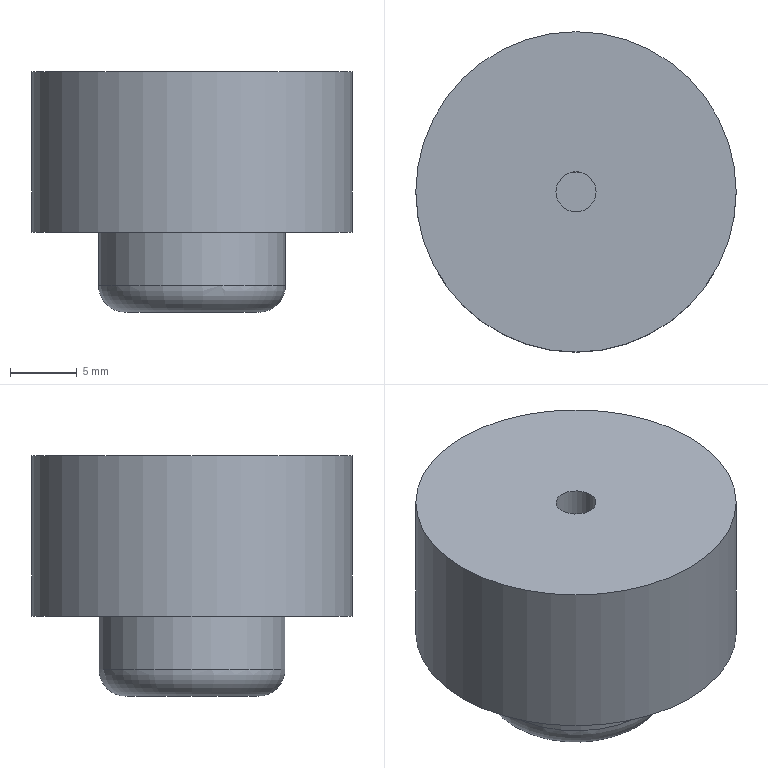Component | NX | MOTOR_MOUNT_3 | 1 solid | 8 faces | box 24 x 24 x 18 mm | volume 6275 mm3 | plane 4 | cylinder 3 | torus 1 | commonest cylinder face diameters 24 x1 14 x1 3 x1
STEP:
#1=CARTESIAN_POINT('',(0.,0.,0.));
#2=DIRECTION('',(0.,0.,1.));
#3=DIRECTION('',(1.,0.,0.));
#4=AXIS2_PLACEMENT_3D('',#1,#2,#3);
#5=CARTESIAN_POINT('',(92.558,84.858,-55.892));
#6=VERTEX_POINT('',#5);
#7=CARTESIAN_POINT('',(85.558,84.858,-55.892));
#8=DIRECTION('',(0.,0.,-1.));
#9=DIRECTION('',(1.,0.,0.));
#10=AXIS2_PLACEMENT_3D('',#7,#8,#9);
#11=CIRCLE('',#10,7.);
#12=CARTESIAN_POINT('',(85.558,84.858,-55.892));
#13=DIRECTION('',(0.,0.,-1.));
#14=DIRECTION('',(1.,0.,0.));
#15=AXIS2_PLACEMENT_3D('',#12,#13,#14);
#16=PLANE('',#15);
#17=CARTESIAN_POINT('',(0.,0.));
#18=DIRECTION('',(1.,0.));
#19=AXIS2_PLACEMENT_2D('',#17,#18);
#20=CIRCLE('',#19,7.);
#21=(GEOMETRIC_REPRESENTATION_CONTEXT(2)PARAMETRIC_REPRESENTATION_CONTEXT()REPRESENTATION_CONTEXT('',''));
#22=DEFINITIONAL_REPRESENTATION('',(#20),#21);
#23=PCURVE('',#16,#22);
#24=CARTESIAN_POINT('',(85.558,84.858,-55.892));
#25=DIRECTION('',(0.,0.,-1.));
#26=DIRECTION('',(1.,0.,0.));
#27=AXIS2_PLACEMENT_3D('',#24,#25,#26);
#28=CYLINDRICAL_SURFACE('',#27,7.);
#29=CARTESIAN_POINT('',(0.,0.));
#30=DIRECTION('',(1.,0.));
#31=VECTOR('',#30,1.);
#32=LINE('',#29,#31);
#33=(GEOMETRIC_REPRESENTATION_CONTEXT(2)PARAMETRIC_REPRESENTATION_CONTEXT()REPRESENTATION_CONTEXT('',''));
#34=DEFINITIONAL_REPRESENTATION('',(#32),#33);
#35=PCURVE('',#28,#34);
#36=SURFACE_CURVE('',#11,(#23,#35),.PCURVE_S1.);
#37=EDGE_CURVE('',#6,#6,#36,.T.);
#38=ORIENTED_EDGE('',*,*,#37,.F.);
#39=EDGE_LOOP('',(#38));
#40=FACE_BOUND('',#39,.T.);
#41=CARTESIAN_POINT('',(97.558,84.858,-55.892));
#42=VERTEX_POINT('',#41);
#43=CARTESIAN_POINT('',(85.558,84.858,-55.892));
#44=DIRECTION('',(0.,0.,1.));
#45=DIRECTION('',(1.,0.,0.));
#46=AXIS2_PLACEMENT_3D('',#43,#44,#45);
#47=CIRCLE('',#46,12.);
#48=CARTESIAN_POINT('',(12.,0.));
#49=CARTESIAN_POINT('',(12.,-20.785));
#50=CARTESIAN_POINT('',(-6.,-10.392));
#51=CARTESIAN_POINT('',(-24.,-0.));
#52=CARTESIAN_POINT('',(-6.,10.392));
#53=CARTESIAN_POINT('',(12.,20.785));
#54=CARTESIAN_POINT('',(12.,0.));
#55=(BOUNDED_CURVE()B_SPLINE_CURVE(2,(#48,#49,#50,#51,#52,#53,#54),.UNSPECIFIED.,.T.,.F.)B_SPLINE_CURVE_WITH_KNOTS((1,2,2,2,2,1),(-2.094,0.,2.094,4.189,6.283,8.378),.UNSPECIFIED.)CURVE()GEOMETRIC_REPRESENTATION_ITEM()RATIONAL_B_SPLINE_CURVE((1.,0.5,1.,0.5,1.,0.5,1.))REPRESENTATION_ITEM(''));
#56=(GEOMETRIC_REPRESENTATION_CONTEXT(2)PARAMETRIC_REPRESENTATION_CONTEXT()REPRESENTATION_CONTEXT('',''));
#57=DEFINITIONAL_REPRESENTATION('',(#55),#56);
#58=PCURVE('',#16,#57);
#59=CARTESIAN_POINT('',(85.558,84.858,-43.892));
#60=DIRECTION('',(0.,0.,-1.));
#61=DIRECTION('',(1.,0.,0.));
#62=AXIS2_PLACEMENT_3D('',#59,#60,#61);
#63=CYLINDRICAL_SURFACE('',#62,12.);
#64=CARTESIAN_POINT('',(6.283,12.));
#65=DIRECTION('',(-1.,0.));
#66=VECTOR('',#65,1.);
#67=LINE('',#64,#66);
#68=(GEOMETRIC_REPRESENTATION_CONTEXT(2)PARAMETRIC_REPRESENTATION_CONTEXT()REPRESENTATION_CONTEXT('',''));
#69=DEFINITIONAL_REPRESENTATION('',(#67),#68);
#70=PCURVE('',#63,#69);
#71=SURFACE_CURVE('',#47,(#58,#70),.PCURVE_S1.);
#72=EDGE_CURVE('',#42,#42,#71,.T.);
#73=ORIENTED_EDGE('',*,*,#72,.F.);
#74=EDGE_LOOP('',(#73));
#75=FACE_BOUND('',#74,.T.);
#76=ADVANCED_FACE('',(#40,#75),#16,.T.);
#77=CARTESIAN_POINT('',(87.058,84.858,-43.892));
#78=VERTEX_POINT('',#77);
#79=CARTESIAN_POINT('',(85.558,84.858,-43.892));
#80=DIRECTION('',(0.,0.,1.));
#81=DIRECTION('',(1.,0.,0.));
#82=AXIS2_PLACEMENT_3D('',#79,#80,#81);
#83=CIRCLE('',#82,1.5);
#84=CARTESIAN_POINT('',(85.558,84.858,-43.892));
#85=DIRECTION('',(0.,0.,1.));
#86=DIRECTION('',(-1.,0.,0.));
#87=AXIS2_PLACEMENT_3D('',#84,#85,#86);
#88=PLANE('',#87);
#89=CARTESIAN_POINT('',(0.,0.));
#90=DIRECTION('',(-1.,0.));
#91=AXIS2_PLACEMENT_2D('',#89,#90);
#92=CIRCLE('',#91,1.5);
#93=(GEOMETRIC_REPRESENTATION_CONTEXT(2)PARAMETRIC_REPRESENTATION_CONTEXT()REPRESENTATION_CONTEXT('',''));
#94=DEFINITIONAL_REPRESENTATION('',(#92),#93);
#95=PCURVE('',#88,#94);
#96=CARTESIAN_POINT('',(85.558,84.858,-49.892));
#97=DIRECTION('',(0.,0.,1.));
#98=DIRECTION('',(-1.,0.,0.));
#99=AXIS2_PLACEMENT_3D('',#96,#97,#98);
#100=CYLINDRICAL_SURFACE('',#99,1.5);
#101=CARTESIAN_POINT('',(3.142,6.));
#102=DIRECTION('',(1.,0.));
#103=VECTOR('',#102,1.);
#104=LINE('',#101,#103);
#105=(GEOMETRIC_REPRESENTATION_CONTEXT(2)PARAMETRIC_REPRESENTATION_CONTEXT()REPRESENTATION_CONTEXT('',''));
#106=DEFINITIONAL_REPRESENTATION('',(#104),#105);
#107=PCURVE('',#100,#106);
#108=SURFACE_CURVE('',#83,(#95,#107),.PCURVE_S1.);
#109=EDGE_CURVE('',#78,#78,#108,.T.);
#110=ORIENTED_EDGE('',*,*,#109,.F.);
#111=EDGE_LOOP('',(#110));
#112=FACE_BOUND('',#111,.T.);
#113=CARTESIAN_POINT('',(97.558,84.858,-43.892));
#114=VERTEX_POINT('',#113);
#115=CARTESIAN_POINT('',(85.558,84.858,-43.892));
#116=DIRECTION('',(0.,0.,-1.));
#117=DIRECTION('',(1.,0.,0.));
#118=AXIS2_PLACEMENT_3D('',#115,#116,#117);
#119=CIRCLE('',#118,12.);
#120=CARTESIAN_POINT('',(-12.,0.));
#121=CARTESIAN_POINT('',(-12.,20.785));
#122=CARTESIAN_POINT('',(6.,10.392));
#123=CARTESIAN_POINT('',(24.,0.));
#124=CARTESIAN_POINT('',(6.,-10.392));
#125=CARTESIAN_POINT('',(-12.,-20.785));
#126=CARTESIAN_POINT('',(-12.,0.));
#127=(BOUNDED_CURVE()B_SPLINE_CURVE(2,(#120,#121,#122,#123,#124,#125,#126),.UNSPECIFIED.,.T.,.F.)B_SPLINE_CURVE_WITH_KNOTS((1,2,2,2,2,1),(-2.094,0.,2.094,4.189,6.283,8.378),.UNSPECIFIED.)CURVE()GEOMETRIC_REPRESENTATION_ITEM()RATIONAL_B_SPLINE_CURVE((1.,0.5,1.,0.5,1.,0.5,1.))REPRESENTATION_ITEM(''));
#128=(GEOMETRIC_REPRESENTATION_CONTEXT(2)PARAMETRIC_REPRESENTATION_CONTEXT()REPRESENTATION_CONTEXT('',''));
#129=DEFINITIONAL_REPRESENTATION('',(#127),#128);
#130=PCURVE('',#88,#129);
#131=CARTESIAN_POINT('',(0.,0.));
#132=DIRECTION('',(1.,0.));
#133=VECTOR('',#132,1.);
#134=LINE('',#131,#133);
#135=(GEOMETRIC_REPRESENTATION_CONTEXT(2)PARAMETRIC_REPRESENTATION_CONTEXT()REPRESENTATION_CONTEXT('',''));
#136=DEFINITIONAL_REPRESENTATION('',(#134),#135);
#137=PCURVE('',#63,#136);
#138=SURFACE_CURVE('',#119,(#130,#137),.PCURVE_S1.);
#139=EDGE_CURVE('',#114,#114,#138,.T.);
#140=ORIENTED_EDGE('',*,*,#139,.F.);
#141=EDGE_LOOP('',(#140));
#142=FACE_BOUND('',#141,.T.);
#143=ADVANCED_FACE('',(#112,#142),#88,.T.);
#144=ORIENTED_EDGE('',*,*,#72,.T.);
#145=CARTESIAN_POINT('',(97.558,84.858,-43.892));
#146=CARTESIAN_POINT('',(97.558,84.858,-55.892));
#147=B_SPLINE_CURVE_WITH_KNOTS('',1,(#145,#146),.UNSPECIFIED.,.F.,.F.,(2,2),(0.,12.),.PIECEWISE_BEZIER_KNOTS.);
#148=CARTESIAN_POINT('',(0.,0.));
#149=DIRECTION('',(0.,1.));
#150=VECTOR('',#149,1.);
#151=LINE('',#148,#150);
#152=(GEOMETRIC_REPRESENTATION_CONTEXT(2)PARAMETRIC_REPRESENTATION_CONTEXT()REPRESENTATION_CONTEXT('',''));
#153=DEFINITIONAL_REPRESENTATION('',(#151),#152);
#154=PCURVE('',#63,#153);
#155=CARTESIAN_POINT('',(6.283,0.));
#156=DIRECTION('',(0.,1.));
#157=VECTOR('',#156,1.);
#158=LINE('',#155,#157);
#159=(GEOMETRIC_REPRESENTATION_CONTEXT(2)PARAMETRIC_REPRESENTATION_CONTEXT()REPRESENTATION_CONTEXT('',''));
#160=DEFINITIONAL_REPRESENTATION('',(#158),#159);
#161=PCURVE('',#63,#160);
#162=SEAM_CURVE('',#147,(#154,#161),.PCURVE_S1.);
#163=EDGE_CURVE('',#114,#42,#162,.T.);
#164=ORIENTED_EDGE('',*,*,#163,.F.);
#165=ORIENTED_EDGE('',*,*,#139,.T.);
#166=ORIENTED_EDGE('',*,*,#163,.T.);
#167=EDGE_LOOP('',(#144,#164,#165,#166));
#168=FACE_BOUND('',#167,.T.);
#169=ADVANCED_FACE('',(#168),#63,.T.);
#170=CARTESIAN_POINT('',(90.558,84.858,-61.892));
#171=VERTEX_POINT('',#170);
#172=CARTESIAN_POINT('',(85.558,84.858,-61.892));
#173=DIRECTION('',(0.,0.,-1.));
#174=DIRECTION('',(1.,0.,0.));
#175=AXIS2_PLACEMENT_3D('',#172,#173,#174);
#176=CIRCLE('',#175,5.);
#177=CARTESIAN_POINT('',(85.558,84.858,-61.892));
#178=DIRECTION('',(0.,0.,-1.));
#179=DIRECTION('',(1.,0.,0.));
#180=AXIS2_PLACEMENT_3D('',#177,#178,#179);
#181=PLANE('',#180);
#182=CARTESIAN_POINT('',(0.,0.));
#183=DIRECTION('',(1.,0.));
#184=AXIS2_PLACEMENT_2D('',#182,#183);
#185=CIRCLE('',#184,5.);
#186=(GEOMETRIC_REPRESENTATION_CONTEXT(2)PARAMETRIC_REPRESENTATION_CONTEXT()REPRESENTATION_CONTEXT('',''));
#187=DEFINITIONAL_REPRESENTATION('',(#185),#186);
#188=PCURVE('',#181,#187);
#189=CARTESIAN_POINT('',(85.558,84.858,-59.892));
#190=DIRECTION('',(0.,0.,-1.));
#191=DIRECTION('',(1.,0.,0.));
#192=AXIS2_PLACEMENT_3D('',#189,#190,#191);
#193=TOROIDAL_SURFACE('',#192,5.,2.);
#194=CARTESIAN_POINT('',(0.,7.854));
#195=DIRECTION('',(1.,0.));
#196=VECTOR('',#195,1.);
#197=LINE('',#194,#196);
#198=(GEOMETRIC_REPRESENTATION_CONTEXT(2)PARAMETRIC_REPRESENTATION_CONTEXT()REPRESENTATION_CONTEXT('',''));
#199=DEFINITIONAL_REPRESENTATION('',(#197),#198);
#200=PCURVE('',#193,#199);
#201=SURFACE_CURVE('',#176,(#188,#200),.PCURVE_S1.);
#202=EDGE_CURVE('',#171,#171,#201,.T.);
#203=ORIENTED_EDGE('',*,*,#202,.T.);
#204=EDGE_LOOP('',(#203));
#205=FACE_BOUND('',#204,.T.);
#206=ADVANCED_FACE('',(#205),#181,.T.);
#207=CARTESIAN_POINT('',(92.558,84.858,-59.892));
#208=VERTEX_POINT('',#207);
#209=CARTESIAN_POINT('',(85.558,84.858,-59.892));
#210=DIRECTION('',(0.,0.,1.));
#211=DIRECTION('',(1.,0.,0.));
#212=AXIS2_PLACEMENT_3D('',#209,#210,#211);
#213=CIRCLE('',#212,7.);
#214=CARTESIAN_POINT('',(6.283,4.));
#215=DIRECTION('',(-1.,0.));
#216=VECTOR('',#215,1.);
#217=LINE('',#214,#216);
#218=(GEOMETRIC_REPRESENTATION_CONTEXT(2)PARAMETRIC_REPRESENTATION_CONTEXT()REPRESENTATION_CONTEXT('',''));
#219=DEFINITIONAL_REPRESENTATION('',(#217),#218);
#220=PCURVE('',#28,#219);
#221=CARTESIAN_POINT('',(6.283,6.283));
#222=DIRECTION('',(-1.,0.));
#223=VECTOR('',#222,1.);
#224=LINE('',#221,#223);
#225=(GEOMETRIC_REPRESENTATION_CONTEXT(2)PARAMETRIC_REPRESENTATION_CONTEXT()REPRESENTATION_CONTEXT('',''));
#226=DEFINITIONAL_REPRESENTATION('',(#224),#225);
#227=PCURVE('',#193,#226);
#228=SURFACE_CURVE('',#213,(#220,#227),.PCURVE_S1.);
#229=EDGE_CURVE('',#208,#208,#228,.T.);
#230=ORIENTED_EDGE('',*,*,#229,.T.);
#231=CARTESIAN_POINT('',(92.558,84.858,-55.892));
#232=CARTESIAN_POINT('',(92.558,84.858,-59.892));
#233=B_SPLINE_CURVE_WITH_KNOTS('',1,(#231,#232),.UNSPECIFIED.,.F.,.F.,(2,2),(0.,4.),.PIECEWISE_BEZIER_KNOTS.);
#234=CARTESIAN_POINT('',(0.,0.));
#235=DIRECTION('',(0.,1.));
#236=VECTOR('',#235,1.);
#237=LINE('',#234,#236);
#238=(GEOMETRIC_REPRESENTATION_CONTEXT(2)PARAMETRIC_REPRESENTATION_CONTEXT()REPRESENTATION_CONTEXT('',''));
#239=DEFINITIONAL_REPRESENTATION('',(#237),#238);
#240=PCURVE('',#28,#239);
#241=CARTESIAN_POINT('',(6.283,0.));
#242=DIRECTION('',(0.,1.));
#243=VECTOR('',#242,1.);
#244=LINE('',#241,#243);
#245=(GEOMETRIC_REPRESENTATION_CONTEXT(2)PARAMETRIC_REPRESENTATION_CONTEXT()REPRESENTATION_CONTEXT('',''));
#246=DEFINITIONAL_REPRESENTATION('',(#244),#245);
#247=PCURVE('',#28,#246);
#248=SEAM_CURVE('',#233,(#240,#247),.PCURVE_S1.);
#249=EDGE_CURVE('',#6,#208,#248,.T.);
#250=ORIENTED_EDGE('',*,*,#249,.F.);
#251=ORIENTED_EDGE('',*,*,#37,.T.);
#252=ORIENTED_EDGE('',*,*,#249,.T.);
#253=EDGE_LOOP('',(#230,#250,#251,#252));
#254=FACE_BOUND('',#253,.T.);
#255=ADVANCED_FACE('',(#254),#28,.T.);
#256=ORIENTED_EDGE('',*,*,#202,.F.);
#257=CARTESIAN_POINT('',(92.558,84.858,-59.892));
#258=CARTESIAN_POINT('',(92.558,84.858,-60.427));
#259=CARTESIAN_POINT('',(92.388,84.858,-60.947));
#260=CARTESIAN_POINT('',(92.062,84.858,-61.396));
#261=CARTESIAN_POINT('',(91.613,84.858,-61.722));
#262=CARTESIAN_POINT('',(91.092,84.858,-61.892));
#263=CARTESIAN_POINT('',(90.558,84.858,-61.892));
#264=(BOUNDED_CURVE()B_SPLINE_CURVE(6,(#257,#258,#259,#260,#261,#262,#263),.UNSPECIFIED.,.F.,.F.)B_SPLINE_CURVE_WITH_KNOTS((7,7),(0.,1.571),.PIECEWISE_BEZIER_KNOTS.)CURVE()GEOMETRIC_REPRESENTATION_ITEM()RATIONAL_B_SPLINE_CURVE((1.031,1.01,0.9979,0.994,0.9979,1.01,1.031))REPRESENTATION_ITEM(''));
#265=CARTESIAN_POINT('',(0.,6.283));
#266=DIRECTION('',(0.,1.));
#267=VECTOR('',#266,1.);
#268=LINE('',#265,#267);
#269=(GEOMETRIC_REPRESENTATION_CONTEXT(2)PARAMETRIC_REPRESENTATION_CONTEXT()REPRESENTATION_CONTEXT('',''));
#270=DEFINITIONAL_REPRESENTATION('',(#268),#269);
#271=PCURVE('',#193,#270);
#272=CARTESIAN_POINT('',(6.283,6.283));
#273=DIRECTION('',(0.,1.));
#274=VECTOR('',#273,1.);
#275=LINE('',#272,#274);
#276=(GEOMETRIC_REPRESENTATION_CONTEXT(2)PARAMETRIC_REPRESENTATION_CONTEXT()REPRESENTATION_CONTEXT('',''));
#277=DEFINITIONAL_REPRESENTATION('',(#275),#276);
#278=PCURVE('',#193,#277);
#279=SEAM_CURVE('',#264,(#271,#278),.PCURVE_S1.);
#280=EDGE_CURVE('',#208,#171,#279,.T.);
#281=ORIENTED_EDGE('',*,*,#280,.F.);
#282=ORIENTED_EDGE('',*,*,#229,.F.);
#283=ORIENTED_EDGE('',*,*,#280,.T.);
#284=EDGE_LOOP('',(#256,#281,#282,#283));
#285=FACE_BOUND('',#284,.T.);
#286=ADVANCED_FACE('',(#285),#193,.T.);
#287=CARTESIAN_POINT('',(87.058,84.858,-49.892));
#288=VERTEX_POINT('',#287);
#289=CARTESIAN_POINT('',(85.558,84.858,-49.892));
#290=DIRECTION('',(0.,0.,-1.));
#291=DIRECTION('',(1.,0.,0.));
#292=AXIS2_PLACEMENT_3D('',#289,#290,#291);
#293=CIRCLE('',#292,1.5);
#294=CARTESIAN_POINT('',(9.425,0.));
#295=DIRECTION('',(-1.,0.));
#296=VECTOR('',#295,1.);
#297=LINE('',#294,#296);
#298=(GEOMETRIC_REPRESENTATION_CONTEXT(2)PARAMETRIC_REPRESENTATION_CONTEXT()REPRESENTATION_CONTEXT('',''));
#299=DEFINITIONAL_REPRESENTATION('',(#297),#298);
#300=PCURVE('',#100,#299);
#301=CARTESIAN_POINT('',(85.558,84.858,-49.892));
#302=DIRECTION('',(0.,0.,1.));
#303=DIRECTION('',(-1.,0.,0.));
#304=AXIS2_PLACEMENT_3D('',#301,#302,#303);
#305=PLANE('',#304);
#306=CARTESIAN_POINT('',(-1.5,0.));
#307=CARTESIAN_POINT('',(-1.5,2.598));
#308=CARTESIAN_POINT('',(0.75,1.299));
#309=CARTESIAN_POINT('',(3.,0.));
#310=CARTESIAN_POINT('',(0.75,-1.299));
#311=CARTESIAN_POINT('',(-1.5,-2.598));
#312=CARTESIAN_POINT('',(-1.5,0.));
#313=(BOUNDED_CURVE()B_SPLINE_CURVE(2,(#306,#307,#308,#309,#310,#311,#312),.UNSPECIFIED.,.T.,.F.)B_SPLINE_CURVE_WITH_KNOTS((1,2,2,2,2,1),(-2.094,0.,2.094,4.189,6.283,8.378),.UNSPECIFIED.)CURVE()GEOMETRIC_REPRESENTATION_ITEM()RATIONAL_B_SPLINE_CURVE((1.,0.5,1.,0.5,1.,0.5,1.))REPRESENTATION_ITEM(''));
#314=(GEOMETRIC_REPRESENTATION_CONTEXT(2)PARAMETRIC_REPRESENTATION_CONTEXT()REPRESENTATION_CONTEXT('',''));
#315=DEFINITIONAL_REPRESENTATION('',(#313),#314);
#316=PCURVE('',#305,#315);
#317=SURFACE_CURVE('',#293,(#300,#316),.PCURVE_S1.);
#318=EDGE_CURVE('',#288,#288,#317,.T.);
#319=ORIENTED_EDGE('',*,*,#318,.F.);
#320=CARTESIAN_POINT('',(87.058,84.858,-49.892));
#321=CARTESIAN_POINT('',(87.058,84.858,-43.892));
#322=B_SPLINE_CURVE_WITH_KNOTS('',1,(#320,#321),.UNSPECIFIED.,.F.,.F.,(2,2),(0.,6.),.PIECEWISE_BEZIER_KNOTS.);
#323=CARTESIAN_POINT('',(9.425,0.));
#324=DIRECTION('',(0.,1.));
#325=VECTOR('',#324,1.);
#326=LINE('',#323,#325);
#327=(GEOMETRIC_REPRESENTATION_CONTEXT(2)PARAMETRIC_REPRESENTATION_CONTEXT()REPRESENTATION_CONTEXT('',''));
#328=DEFINITIONAL_REPRESENTATION('',(#326),#327);
#329=PCURVE('',#100,#328);
#330=CARTESIAN_POINT('',(3.142,0.));
#331=DIRECTION('',(0.,1.));
#332=VECTOR('',#331,1.);
#333=LINE('',#330,#332);
#334=(GEOMETRIC_REPRESENTATION_CONTEXT(2)PARAMETRIC_REPRESENTATION_CONTEXT()REPRESENTATION_CONTEXT('',''));
#335=DEFINITIONAL_REPRESENTATION('',(#333),#334);
#336=PCURVE('',#100,#335);
#337=SEAM_CURVE('',#322,(#329,#336),.PCURVE_S1.);
#338=EDGE_CURVE('',#288,#78,#337,.T.);
#339=ORIENTED_EDGE('',*,*,#338,.T.);
#340=ORIENTED_EDGE('',*,*,#109,.F.);
#341=ORIENTED_EDGE('',*,*,#338,.F.);
#342=EDGE_LOOP('',(#319,#339,#340,#341));
#343=FACE_BOUND('',#342,.F.);
#344=ADVANCED_FACE('',(#343),#100,.F.);
#345=ORIENTED_EDGE('',*,*,#318,.F.);
#346=EDGE_LOOP('',(#345));
#347=FACE_BOUND('',#346,.T.);
#348=ADVANCED_FACE('',(#347),#305,.T.);
#349=CLOSED_SHELL('',(#76,#143,#169,#206,#255,#286,#344,#348));
#350=MANIFOLD_SOLID_BREP('',#349);
#351=(LENGTH_UNIT()NAMED_UNIT(*)SI_UNIT(.MILLI.,.METRE.));
#352=UNCERTAINTY_MEASURE_WITH_UNIT(LENGTH_MEASURE(0.00001),#351,'','');
#353=(NAMED_UNIT(*)PLANE_ANGLE_UNIT()SI_UNIT($,.RADIAN.));
#354=(NAMED_UNIT(*)SI_UNIT($,.STERADIAN.)SOLID_ANGLE_UNIT());
#355=(GEOMETRIC_REPRESENTATION_CONTEXT(3)GLOBAL_UNCERTAINTY_ASSIGNED_CONTEXT((#352))GLOBAL_UNIT_ASSIGNED_CONTEXT((#351,#353,#354))REPRESENTATION_CONTEXT('',''));
#356=ADVANCED_BREP_SHAPE_REPRESENTATION('',(#4,#350),#355);